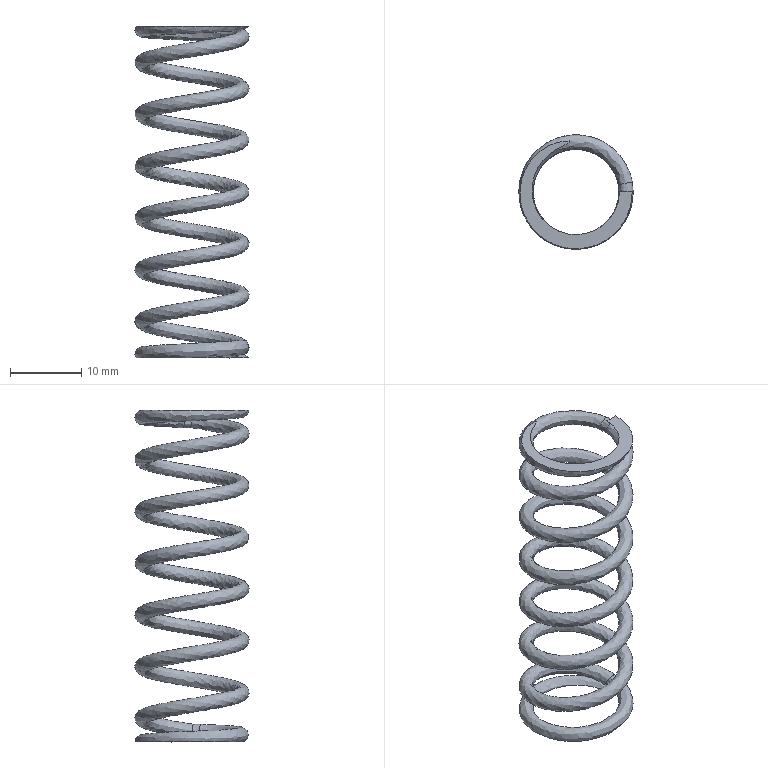Component | NX | SPRING | 1 solid | 9 faces | volume 1056 mm3 | spline 5 | plane 4